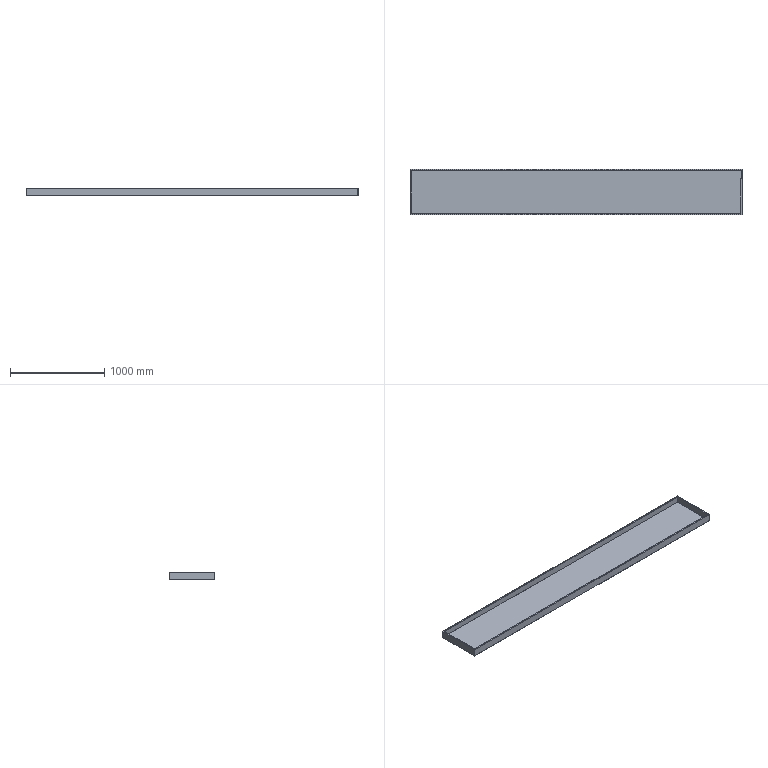Component | NX | DB5 | 1 solid | 17 faces | volume 3639616 mm3 | plane 17